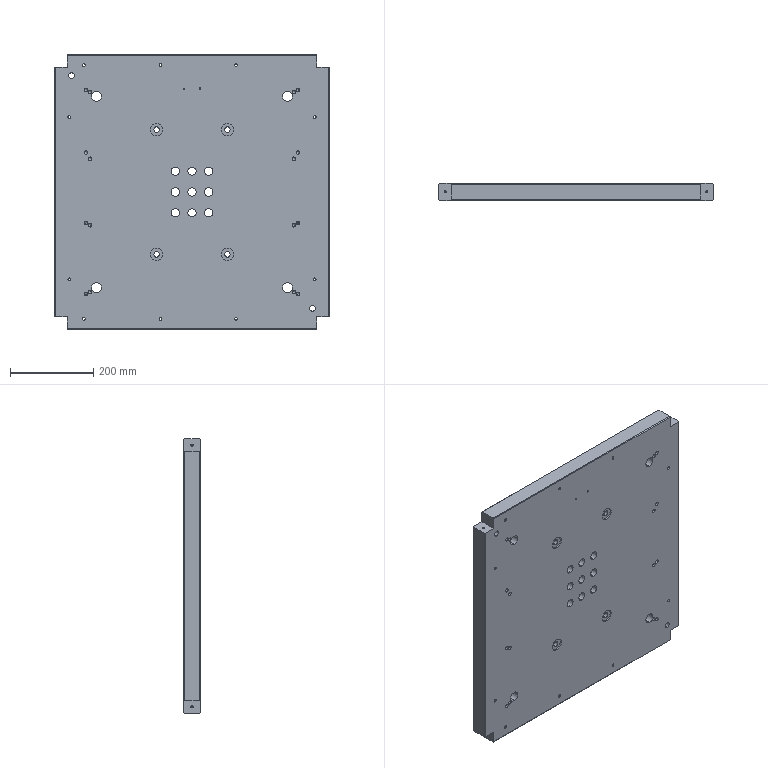Component | SolidWorks | Plate1-2 | 1 solid | 494 faces | box 660 x 40 x 660 mm | volume 16935087 mm3 | cylinder 274 | cone 180 | plane 40 | commonest cylinder face diameters 8.5 x128 5 x40 20 x26 11 x20 6.6 x20 2.5 x8 13.5 x8 30 x8
build123d program:
from build123d import *

# Parameters (mm, degrees)
SKETCH1_W                                        = 660
SKETCH1_H                                        = 660
BOSS_EXTRUDE1_DEPTH                              = 40
SKETCH2_R                                        = 12
CUT_EXTRUDE1_DEPTH                               = 935.238
SKETCH3_R                                        = 15
CUT_EXTRUDE2_DEPTH                               = 4
M16_TAPPED_HOLE1_D                               = 14
M12_HEX_SOCKET_HEAD_CAP_SCREW_CBORE1_D           = 13.5
M12_HEX_SOCKET_HEAD_CAP_SCREW_CBORE1_CBORE_D     = 20
M12_HEX_SOCKET_HEAD_CAP_SCREW_CBORE1_CBORE_DEPTH = 12.6
M12_HEX_SOCKET_HEAD_CAP_SCREW_CBORE2_D           = 13.5
M12_HEX_SOCKET_HEAD_CAP_SCREW_CBORE2_CBORE_D     = 20
M12_HEX_SOCKET_HEAD_CAP_SCREW_CBORE2_CBORE_DEPTH = 12.6
CHAMFER1_SIZE                                    = 5
CHAMFER2_SIZE                                    = 2
M4_TAPPED_HOLE2_D                                = 3.3
M4_TAPPED_HOLE2_DEPTH                            = 15.5
M4_TAPPED_HOLE2_TIP                              = 0.9914
SKETCH18_W                                       = 49.476
SKETCH18_H                                       = 71.934
SKETCH18_W_2                                     = 85.581
SKETCH18_H_2                                     = 93.055
SKETCH18_W_3                                     = 57.475
SKETCH18_H_3                                     = 122.53
SKETCH18_W_4                                     = 110.229
SKETCH18_H_4                                     = 53.292
CUT_EXTRUDE3_DEPTH                               = 935.238
M6_TAPPED_HOLE1_D                                = 5
M6_TAPPED_HOLE1_DEPTH                            = 17
M6_TAPPED_HOLE1_TIP                              = 1.502
M6_TAPPED_HOLE2_D                                = 5
M6_TAPPED_HOLE2_DEPTH                            = 17
M6_TAPPED_HOLE2_TIP                              = 1.502
M6_HEX_SOCKET_HEAD_CAP_SCREW_CBORE1_D            = 6.6
M6_HEX_SOCKET_HEAD_CAP_SCREW_CBORE1_CBORE_D      = 11
M6_HEX_SOCKET_HEAD_CAP_SCREW_CBORE1_CBORE_DEPTH  = 6.4
M6_HEX_SOCKET_HEAD_CAP_SCREW_CBORE2_D            = 6.6
M6_HEX_SOCKET_HEAD_CAP_SCREW_CBORE2_CBORE_D      = 11
M6_HEX_SOCKET_HEAD_CAP_SCREW_CBORE2_CBORE_DEPTH  = 6.4
M10_TAPPED_HOLE1_D                               = 8.5
M10_TAPPED_HOLE1_DEPTH                           = 20
M10_TAPPED_HOLE1_TIP                             = 2.554
M6_TAPPED_HOLE3_D                                = 5
M6_TAPPED_HOLE3_DEPTH                            = 15
M6_TAPPED_HOLE3_TIP                              = 1.502
M6_TAPPED_HOLE4_D                                = 5
M6_TAPPED_HOLE4_DEPTH                            = 16
M6_TAPPED_HOLE4_TIP                              = 1.502
M3_TAPPED_HOLE1_D                                = 2.5
M3_TAPPED_HOLE1_DEPTH                            = 8.5
M3_TAPPED_HOLE1_TIP                              = 0.7511
M6_TAPPED_HOLE5_D                                = 5
M6_TAPPED_HOLE5_DEPTH                            = 17
M6_TAPPED_HOLE5_TIP                              = 1.502
M6_TAPPED_HOLE6_D                                = 5
M6_TAPPED_HOLE6_DEPTH                            = 17
M6_TAPPED_HOLE6_TIP                              = 1.502
M6_TAPPED_HOLE7_D                                = 5
M6_TAPPED_HOLE7_DEPTH                            = 17
M6_TAPPED_HOLE7_TIP                              = 1.502
M10_TAPPED_HOLE2_D                               = 8.5
M10_TAPPED_HOLE2_DEPTH                           = 18
M10_TAPPED_HOLE2_TIP                             = 2.554
SKETCH49_R                                       = 10
CUT_EXTRUDE4_DEPTH                               = 935.238
M10_TAPPED_HOLE3_D                               = 8.5
M10_TAPPED_HOLE3_DEPTH                           = 24.5
M10_TAPPED_HOLE3_TIP                             = 2.554


with BuildPart() as part:
    # Sketch1 → Boss-Extrude1 (new body)
    with BuildSketch(Plane.XY):
        with Locations((330, 330)):
            Rectangle(SKETCH1_W, SKETCH1_H)
    extrude(amount=BOSS_EXTRUDE1_DEPTH)

    # Sketch2 → Cut-Extrude1 (cut, through all)
    with BuildSketch(Plane.XY.offset(40)):
        with Locations((100, 100)):
            Circle(SKETCH2_R)
        with Locations((100, 560)):
            Circle(SKETCH2_R)
        with Locations((560, 560)):
            Circle(SKETCH2_R)
        with Locations((560, 100)):
            Circle(SKETCH2_R)
    extrude(amount=-CUT_EXTRUDE1_DEPTH, mode=Mode.SUBTRACT)

    # Sketch3 → Cut-Extrude2 (cut)
    with BuildSketch(Plane(origin=(0, 0, 0), x_dir=(-1, 0, 0), z_dir=(0, 0, -1))):
        with Locations((-480, 245)):
            Circle(SKETCH3_R)
        with Locations(Location((-480, 415, 0), (0, 0, 180))):
            Circle(SKETCH3_R)
        with Locations((-180, 415)):
            Circle(SKETCH3_R)
        with Locations(Location((-180, 245, 0), (0, 0, 180))):
            Circle(SKETCH3_R)
    extrude(amount=-CUT_EXTRUDE2_DEPTH, mode=Mode.SUBTRACT)

    # M16 Tapped Hole1 (through all)
    with Locations(Plane.XY.offset(40)):
        with Locations((50, 620), (610, 40)):
            Hole(M16_TAPPED_HOLE1_D / 2)

    # M12 Hex Socket Head Cap Screw CBORE1 (through all)
    with Locations(Plane.XY.offset(40)):
        with Locations((480, 415), (480, 245)):
            CounterBoreHole(M12_HEX_SOCKET_HEAD_CAP_SCREW_CBORE1_D / 2, M12_HEX_SOCKET_HEAD_CAP_SCREW_CBORE1_CBORE_D / 2, M12_HEX_SOCKET_HEAD_CAP_SCREW_CBORE1_CBORE_DEPTH)

    # M12 Hex Socket Head Cap Screw CBORE2 (through all)
    with Locations(Plane.XY.offset(40)):
        with Locations((180, 415), (180, 245)):
            CounterBoreHole(M12_HEX_SOCKET_HEAD_CAP_SCREW_CBORE2_D / 2, M12_HEX_SOCKET_HEAD_CAP_SCREW_CBORE2_CBORE_D / 2, M12_HEX_SOCKET_HEAD_CAP_SCREW_CBORE2_CBORE_DEPTH)

    # Chamfer1
    chamfer1_edges = [part.edges().sort_by_distance(p)[0] for p in [
        (0, 660, 20),
        (660, 660, 20),
        (660, 0, 20),
        (0, 0, 20),
    ]]
    chamfer(chamfer1_edges, length=CHAMFER1_SIZE)

    # Chamfer2
    chamfer2_edges = [part.edges().sort_by_distance(p)[0] for p in [
        (660, 330, 40),
        (0, 330, 40),
        (330, 0, 40),
        (330, 660, 0),
        (330, 660, 40),
        (0, 330, 0),
        (660, 330, 0),
        (330, 0, 0),
    ]]
    chamfer(chamfer2_edges, length=CHAMFER2_SIZE)

    # M4 Tapped Hole2
    with Locations(Plane(origin=(0, 0, 0), x_dir=(-1, 0, 0), z_dir=(0, 0, -1))):
        with Locations((-82.5, 350), (-81.185, 310)):
            Hole(M4_TAPPED_HOLE2_D / 2, depth=M4_TAPPED_HOLE2_DEPTH)
            with Locations((0, 0, -(M4_TAPPED_HOLE2_DEPTH + M4_TAPPED_HOLE2_TIP / 2))):  # 118° drill point
                Cone(0, M4_TAPPED_HOLE2_D / 2, M4_TAPPED_HOLE2_TIP, mode=Mode.SUBTRACT)

    # Sketch18 → Cut-Extrude3 (cut, through all)
    with BuildSketch(Plane.XY.offset(40)):
        with Locations((5.262, 665.967)):
            Rectangle(SKETCH18_W, SKETCH18_H)
        with Locations((-12.791, -16.528)):
            Rectangle(SKETCH18_W_2, SKETCH18_H_2)
        with Locations((658.738, -31.265)):
            Rectangle(SKETCH18_W_3, SKETCH18_H_3)
        with Locations((685.114, 656.646)):
            Rectangle(SKETCH18_W_4, SKETCH18_H_4)
    extrude(amount=-CUT_EXTRUDE3_DEPTH, mode=Mode.SUBTRACT)

    # M6 Tapped Hole1
    with Locations(Plane(origin=(630, 0, 0), x_dir=(0, 0, -1), z_dir=(1, 0, 0))):
        with Locations((-20, 15), (-20, 645)):
            Hole(M6_TAPPED_HOLE1_D / 2, depth=M6_TAPPED_HOLE1_DEPTH)
            with Locations((0, 0, -(M6_TAPPED_HOLE1_DEPTH + M6_TAPPED_HOLE1_TIP / 2))):  # 118° drill point
                Cone(0, M6_TAPPED_HOLE1_D / 2, M6_TAPPED_HOLE1_TIP, mode=Mode.SUBTRACT)

    # M6 Tapped Hole2
    with Locations(Plane.ZY.offset(-30)):
        with Locations((20, 645), (20, 15)):
            Hole(M6_TAPPED_HOLE2_D / 2, depth=M6_TAPPED_HOLE2_DEPTH)
            with Locations((0, 0, -(M6_TAPPED_HOLE2_DEPTH + M6_TAPPED_HOLE2_TIP / 2))):  # 118° drill point
                Cone(0, M6_TAPPED_HOLE2_D / 2, M6_TAPPED_HOLE2_TIP, mode=Mode.SUBTRACT)

    # M6 Hex Socket Head Cap Screw CBORE1 (through all)
    with Locations(Plane.XY.offset(40)):
        with Locations((150, 35), (540, 35), (540, 625), (150, 625)):
            CounterBoreHole(M6_HEX_SOCKET_HEAD_CAP_SCREW_CBORE1_D / 2, M6_HEX_SOCKET_HEAD_CAP_SCREW_CBORE1_CBORE_D / 2, M6_HEX_SOCKET_HEAD_CAP_SCREW_CBORE1_CBORE_DEPTH)

    # M6 Hex Socket Head Cap Screw CBORE2 (through all)
    with Locations(Plane.XY.offset(40)):
        with Locations((25, 590), (25, 224.136), (635, 590), (635, 405.91), (635, 224.136), (25, 405.91)):
            CounterBoreHole(M6_HEX_SOCKET_HEAD_CAP_SCREW_CBORE2_D / 2, M6_HEX_SOCKET_HEAD_CAP_SCREW_CBORE2_CBORE_D / 2, M6_HEX_SOCKET_HEAD_CAP_SCREW_CBORE2_CBORE_DEPTH)

    # M10 Tapped Hole1
    with Locations(Plane(origin=(0, 0, 0), x_dir=(-1, 0, 0), z_dir=(0, 0, -1))):
        with Locations((-90, 575), (-250, 575), (-410, 575), (-570, 575), (-570, 85), (-410, 85), (-250, 85), (-90, 85)):
            Hole(M10_TAPPED_HOLE1_D / 2, depth=M10_TAPPED_HOLE1_DEPTH)
            with Locations((0, 0, -(M10_TAPPED_HOLE1_DEPTH + M10_TAPPED_HOLE1_TIP / 2))):  # 118° drill point
                Cone(0, M10_TAPPED_HOLE1_D / 2, M10_TAPPED_HOLE1_TIP, mode=Mode.SUBTRACT)

    # M6 Tapped Hole3
    with Locations(Plane.XY.offset(40)):
        with Locations((575, 191), (645, 191), (575, 469), (645, 469)):
            Hole(M6_TAPPED_HOLE3_D / 2, depth=M6_TAPPED_HOLE3_DEPTH)
            with Locations((0, 0, -(M6_TAPPED_HOLE3_DEPTH + M6_TAPPED_HOLE3_TIP / 2))):  # 118° drill point
                Cone(0, M6_TAPPED_HOLE3_D / 2, M6_TAPPED_HOLE3_TIP, mode=Mode.SUBTRACT)

    # M6 Tapped Hole4
    with Locations(Plane.XY.offset(40)):
        with Locations((85, 469), (15, 469), (85, 191), (15, 191)):
            Hole(M6_TAPPED_HOLE4_D / 2, depth=M6_TAPPED_HOLE4_DEPTH)
            with Locations((0, 0, -(M6_TAPPED_HOLE4_DEPTH + M6_TAPPED_HOLE4_TIP / 2))):  # 118° drill point
                Cone(0, M6_TAPPED_HOLE4_D / 2, M6_TAPPED_HOLE4_TIP, mode=Mode.SUBTRACT)

    # M3 Tapped Hole1
    with Locations(Plane.XY.offset(40)):
        with Locations((569.25, 30.866), (614.25, 30.866), (45.75, 632.269), (90.75, 632.269)):
            Hole(M3_TAPPED_HOLE1_D / 2, depth=M3_TAPPED_HOLE1_DEPTH)
            with Locations((0, 0, -(M3_TAPPED_HOLE1_DEPTH + M3_TAPPED_HOLE1_TIP / 2))):  # 118° drill point
                Cone(0, M3_TAPPED_HOLE1_D / 2, M3_TAPPED_HOLE1_TIP, mode=Mode.SUBTRACT)

    # M6 Tapped Hole5
    with Locations(Plane.XY.offset(40)):
        with Locations((14, 610), (14, 50), (646, 50), (646, 610)):
            Hole(M6_TAPPED_HOLE5_D / 2, depth=M6_TAPPED_HOLE5_DEPTH)
            with Locations((0, 0, -(M6_TAPPED_HOLE5_DEPTH + M6_TAPPED_HOLE5_TIP / 2))):  # 118° drill point
                Cone(0, M6_TAPPED_HOLE5_D / 2, M6_TAPPED_HOLE5_TIP, mode=Mode.SUBTRACT)

    # M6 Tapped Hole6
    with Locations(Plane(origin=(0, 30, 0), x_dir=(-1, 0, 0), z_dir=(0, -1, 0))):
        with Locations((-15, -20), (-645, -20)):
            Hole(M6_TAPPED_HOLE6_D / 2, depth=M6_TAPPED_HOLE6_DEPTH)
            with Locations((0, 0, -(M6_TAPPED_HOLE6_DEPTH + M6_TAPPED_HOLE6_TIP / 2))):  # 118° drill point
                Cone(0, M6_TAPPED_HOLE6_D / 2, M6_TAPPED_HOLE6_TIP, mode=Mode.SUBTRACT)

    # M6 Tapped Hole7
    with Locations(Plane(origin=(0, 630, 0), x_dir=(1, 0, 0), z_dir=(0, 1, 0))):
        with Locations((15, -20), (645, -20)):
            Hole(M6_TAPPED_HOLE7_D / 2, depth=M6_TAPPED_HOLE7_DEPTH)
            with Locations((0, 0, -(M6_TAPPED_HOLE7_DEPTH + M6_TAPPED_HOLE7_TIP / 2))):  # 118° drill point
                Cone(0, M6_TAPPED_HOLE7_D / 2, M6_TAPPED_HOLE7_TIP, mode=Mode.SUBTRACT)

    # M10 Tapped Hole2
    with Locations(Plane.XY.offset(40)):
        with Locations((210, 190), (250, 190), (270, 190), (390, 190), (410, 190), (430, 190), (430, 230), (430, 150), (410, 150), (410, 230), (390, 230), (390, 150), (270, 150), (270, 230), (250, 230), (250, 150), (230, 150), (210, 230), (210, 150), (450, 150), (230, 190), (230, 230), (450, 230), (450, 190), (450, 470), (450, 430), (230, 430), (230, 470), (450, 510), (210, 510), (210, 430), (230, 510), (250, 510), (250, 430), (270, 430), (270, 510), (390, 510), (390, 430), (410, 430), (410, 510), (430, 510), (430, 430), (430, 470), (410, 470), (390, 470), (270, 470), (250, 470), (210, 470)):
            Hole(M10_TAPPED_HOLE2_D / 2, depth=M10_TAPPED_HOLE2_DEPTH)
            with Locations((0, 0, -(M10_TAPPED_HOLE2_DEPTH + M10_TAPPED_HOLE2_TIP / 2))):  # 118° drill point
                Cone(0, M10_TAPPED_HOLE2_D / 2, M10_TAPPED_HOLE2_TIP, mode=Mode.SUBTRACT)

    # Sketch49 → Cut-Extrude4 (cut, through all)
    with BuildSketch(Plane.XY.offset(40)):
        with Locations((330, 330)):
            Circle(SKETCH49_R)
        with Locations((380, 330)):
            Circle(SKETCH49_R)
        with Locations((280, 330)):
            Circle(SKETCH49_R)
        with Locations(Location((380, 370, 0), (0, 0, 180))):
            Circle(SKETCH49_R)
        with Locations(Location((330, 370, 0), (0, 0, 180))):
            Circle(SKETCH49_R)
        with Locations(Location((280, 370, 0), (0, 0, 180))):
            Circle(SKETCH49_R)
        with Locations((280, 290)):
            Circle(SKETCH49_R)
        with Locations((330, 290)):
            Circle(SKETCH49_R)
        with Locations((380, 290)):
            Circle(SKETCH49_R)
    extrude(amount=-CUT_EXTRUDE4_DEPTH, mode=Mode.SUBTRACT)

    # M10 Tapped Hole3
    with Locations(Plane(origin=(0, 0, 0), x_dir=(-1, 0, 0), z_dir=(0, 0, -1))):
        with Locations((-575, 585), (-405, 585), (-235, 585), (-85, 585), (-85, 75), (-235, 75), (-405, 75), (-575, 75)):
            Hole(M10_TAPPED_HOLE3_D / 2, depth=M10_TAPPED_HOLE3_DEPTH)
            with Locations((0, 0, -(M10_TAPPED_HOLE3_DEPTH + M10_TAPPED_HOLE3_TIP / 2))):  # 118° drill point
                Cone(0, M10_TAPPED_HOLE3_D / 2, M10_TAPPED_HOLE3_TIP, mode=Mode.SUBTRACT)


solid = part.part

# Placed as in the assembly
solid = solid.moved(Location((152.049, 277.323, 335), (-90, 0, 90)))